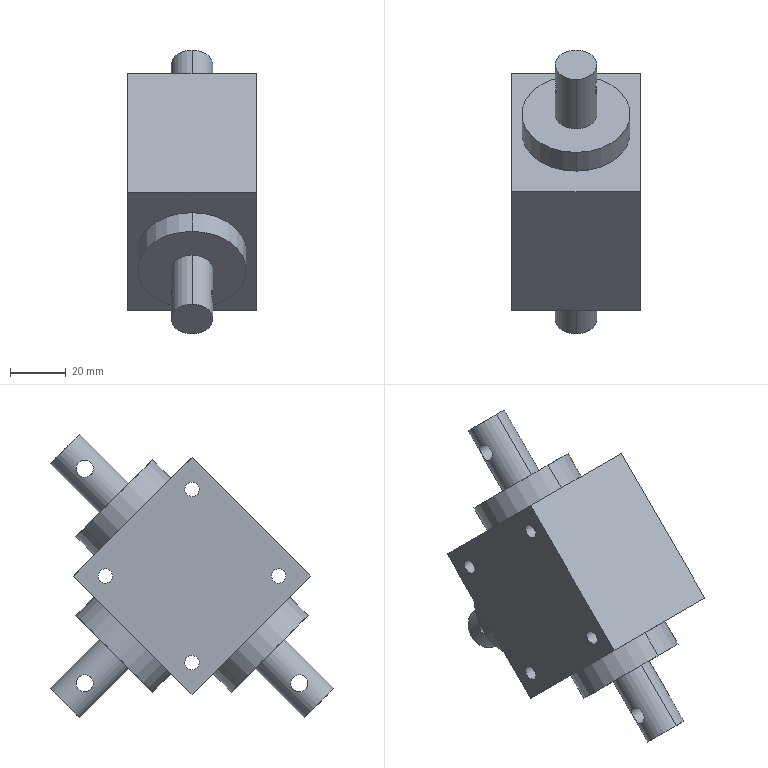Component | SolidWorks | AssemblyDriveAxis-1_1520F-T-1 | 1 solid | 50 faces | volume 205325 mm3 | cylinder 34 | plane 16 | commonest cylinder face diameters 5.2 x8 11 x8 15 x6 6.2 x6 39 x4 39.008 x2